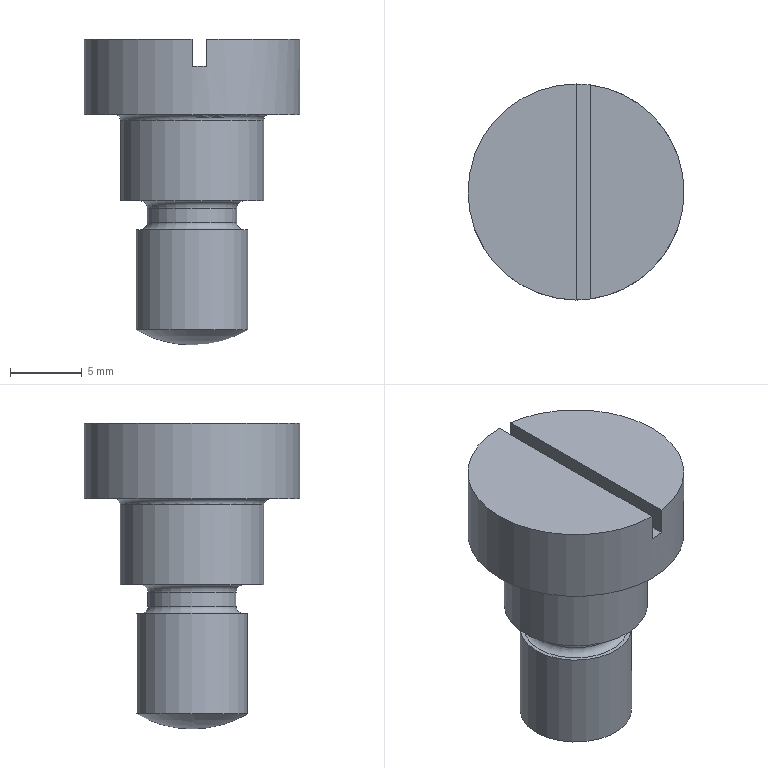Component | NX | GB830-88_M8X6 | 1 solid | 16 faces | box 15 x 15 x 21.24 mm | volume 1783 mm3 | plane 8 | cylinder 4 | torus 3 | sphere 1 | commonest cylinder face diameters 15 x1 9.96 x1 6.2 x1 7.76 x1
STEP:
#1=CARTESIAN_POINT('',(0.,0.,0.));
#2=DIRECTION('',(0.,0.,1.));
#3=DIRECTION('',(1.,0.,0.));
#4=AXIS2_PLACEMENT_3D('',#1,#2,#3);
#5=CARTESIAN_POINT('',(-6.,-7.433,106.24));
#6=VERTEX_POINT('',#5);
#7=CARTESIAN_POINT('',(-6.,7.433,106.24));
#8=VERTEX_POINT('',#7);
#9=CARTESIAN_POINT('',(-6.,-7.5,106.24));
#10=DIRECTION('',(0.,1.,0.));
#11=VECTOR('',#10,1.);
#12=LINE('',#9,#11);
#13=CARTESIAN_POINT('',(0.5,-0.,106.24));
#14=DIRECTION('',(0.,0.,-1.));
#15=DIRECTION('',(-1.,0.,0.));
#16=AXIS2_PLACEMENT_3D('',#13,#14,#15);
#17=PLANE('',#16);
#18=CARTESIAN_POINT('',(6.5,-7.5));
#19=DIRECTION('',(0.,1.));
#20=VECTOR('',#19,1.);
#21=LINE('',#18,#20);
#22=(GEOMETRIC_REPRESENTATION_CONTEXT(2)PARAMETRIC_REPRESENTATION_CONTEXT()REPRESENTATION_CONTEXT('',''));
#23=DEFINITIONAL_REPRESENTATION('',(#21),#22);
#24=PCURVE('',#17,#23);
#25=CARTESIAN_POINT('',(-6.,-7.5,104.34));
#26=DIRECTION('',(-1.,0.,-0.));
#27=DIRECTION('',(-0.,0.,1.));
#28=AXIS2_PLACEMENT_3D('',#25,#26,#27);
#29=PLANE('',#28);
#30=CARTESIAN_POINT('',(1.9,0.));
#31=DIRECTION('',(0.,1.));
#32=VECTOR('',#31,1.);
#33=LINE('',#30,#32);
#34=(GEOMETRIC_REPRESENTATION_CONTEXT(2)PARAMETRIC_REPRESENTATION_CONTEXT()REPRESENTATION_CONTEXT('',''));
#35=DEFINITIONAL_REPRESENTATION('',(#33),#34);
#36=PCURVE('',#29,#35);
#37=SURFACE_CURVE('',#12,(#24,#36),.PCURVE_S1.);
#38=EDGE_CURVE('',#6,#8,#37,.T.);
#39=ORIENTED_EDGE('',*,*,#38,.F.);
#40=CARTESIAN_POINT('',(0.5,-0.,106.24));
#41=VERTEX_POINT('',#40);
#42=CARTESIAN_POINT('',(-7.,-0.,106.24));
#43=DIRECTION('',(0.,0.,1.));
#44=DIRECTION('',(1.,0.,0.));
#45=AXIS2_PLACEMENT_3D('',#42,#43,#44);
#46=CIRCLE('',#45,7.5);
#47=CARTESIAN_POINT('',(0.,0.));
#48=CARTESIAN_POINT('',(0.,12.99));
#49=CARTESIAN_POINT('',(11.25,6.495));
#50=CARTESIAN_POINT('',(22.5,0.));
#51=CARTESIAN_POINT('',(11.25,-6.495));
#52=CARTESIAN_POINT('',(0.,-12.99));
#53=CARTESIAN_POINT('',(0.,0.));
#54=(BOUNDED_CURVE()B_SPLINE_CURVE(2,(#47,#48,#49,#50,#51,#52,#53),.UNSPECIFIED.,.T.,.F.)B_SPLINE_CURVE_WITH_KNOTS((1,2,2,2,2,1),(-2.094,0.,2.094,4.189,6.283,8.378),.UNSPECIFIED.)CURVE()GEOMETRIC_REPRESENTATION_ITEM()RATIONAL_B_SPLINE_CURVE((1.,0.5,1.,0.5,1.,0.5,1.))REPRESENTATION_ITEM(''));
#55=(GEOMETRIC_REPRESENTATION_CONTEXT(2)PARAMETRIC_REPRESENTATION_CONTEXT()REPRESENTATION_CONTEXT('',''));
#56=DEFINITIONAL_REPRESENTATION('',(#54),#55);
#57=PCURVE('',#17,#56);
#58=CARTESIAN_POINT('',(-7.,-0.,101.));
#59=DIRECTION('',(0.,0.,1.));
#60=DIRECTION('',(1.,0.,0.));
#61=AXIS2_PLACEMENT_3D('',#58,#59,#60);
#62=CYLINDRICAL_SURFACE('',#61,7.5);
#63=CARTESIAN_POINT('',(0.,5.24));
#64=DIRECTION('',(1.,0.));
#65=VECTOR('',#64,1.);
#66=LINE('',#63,#65);
#67=(GEOMETRIC_REPRESENTATION_CONTEXT(2)PARAMETRIC_REPRESENTATION_CONTEXT()REPRESENTATION_CONTEXT('',''));
#68=DEFINITIONAL_REPRESENTATION('',(#66),#67);
#69=PCURVE('',#62,#68);
#70=SURFACE_CURVE('',#46,(#57,#69),.PCURVE_S1.);
#71=EDGE_CURVE('',#6,#41,#70,.T.);
#72=ORIENTED_EDGE('',*,*,#71,.T.);
#73=CARTESIAN_POINT('',(-7.,-0.,106.24));
#74=DIRECTION('',(0.,0.,1.));
#75=DIRECTION('',(1.,0.,0.));
#76=AXIS2_PLACEMENT_3D('',#73,#74,#75);
#77=CIRCLE('',#76,7.5);
#78=CARTESIAN_POINT('',(0.,0.));
#79=CARTESIAN_POINT('',(0.,12.99));
#80=CARTESIAN_POINT('',(11.25,6.495));
#81=CARTESIAN_POINT('',(22.5,0.));
#82=CARTESIAN_POINT('',(11.25,-6.495));
#83=CARTESIAN_POINT('',(0.,-12.99));
#84=CARTESIAN_POINT('',(0.,0.));
#85=(BOUNDED_CURVE()B_SPLINE_CURVE(2,(#78,#79,#80,#81,#82,#83,#84),.UNSPECIFIED.,.T.,.F.)B_SPLINE_CURVE_WITH_KNOTS((1,2,2,2,2,1),(-2.094,0.,2.094,4.189,6.283,8.378),.UNSPECIFIED.)CURVE()GEOMETRIC_REPRESENTATION_ITEM()RATIONAL_B_SPLINE_CURVE((1.,0.5,1.,0.5,1.,0.5,1.))REPRESENTATION_ITEM(''));
#86=(GEOMETRIC_REPRESENTATION_CONTEXT(2)PARAMETRIC_REPRESENTATION_CONTEXT()REPRESENTATION_CONTEXT('',''));
#87=DEFINITIONAL_REPRESENTATION('',(#85),#86);
#88=PCURVE('',#17,#87);
#89=CARTESIAN_POINT('',(-6.283,5.24));
#90=DIRECTION('',(1.,0.));
#91=VECTOR('',#90,1.);
#92=LINE('',#89,#91);
#93=(GEOMETRIC_REPRESENTATION_CONTEXT(2)PARAMETRIC_REPRESENTATION_CONTEXT()REPRESENTATION_CONTEXT('',''));
#94=DEFINITIONAL_REPRESENTATION('',(#92),#93);
#95=PCURVE('',#62,#94);
#96=SURFACE_CURVE('',#77,(#88,#95),.PCURVE_S1.);
#97=EDGE_CURVE('',#41,#8,#96,.T.);
#98=ORIENTED_EDGE('',*,*,#97,.T.);
#99=EDGE_LOOP('',(#39,#72,#98));
#100=FACE_BOUND('',#99,.T.);
#101=ADVANCED_FACE('',(#100),#17,.F.);
#102=CARTESIAN_POINT('',(0.5,-0.,101.));
#103=VERTEX_POINT('',#102);
#104=CARTESIAN_POINT('',(-7.,-0.,101.));
#105=DIRECTION('',(0.,0.,1.));
#106=DIRECTION('',(1.,0.,0.));
#107=AXIS2_PLACEMENT_3D('',#104,#105,#106);
#108=CIRCLE('',#107,7.5);
#109=CARTESIAN_POINT('',(0.,0.));
#110=DIRECTION('',(1.,0.));
#111=VECTOR('',#110,1.);
#112=LINE('',#109,#111);
#113=(GEOMETRIC_REPRESENTATION_CONTEXT(2)PARAMETRIC_REPRESENTATION_CONTEXT()REPRESENTATION_CONTEXT('',''));
#114=DEFINITIONAL_REPRESENTATION('',(#112),#113);
#115=PCURVE('',#62,#114);
#116=CARTESIAN_POINT('',(-2.02,-0.,101.));
#117=DIRECTION('',(0.,0.,1.));
#118=DIRECTION('',(1.,0.,0.));
#119=AXIS2_PLACEMENT_3D('',#116,#117,#118);
#120=PLANE('',#119);
#121=CARTESIAN_POINT('',(-4.98,0.));
#122=DIRECTION('',(1.,0.));
#123=AXIS2_PLACEMENT_2D('',#121,#122);
#124=CIRCLE('',#123,7.5);
#125=(GEOMETRIC_REPRESENTATION_CONTEXT(2)PARAMETRIC_REPRESENTATION_CONTEXT()REPRESENTATION_CONTEXT('',''));
#126=DEFINITIONAL_REPRESENTATION('',(#124),#125);
#127=PCURVE('',#120,#126);
#128=SURFACE_CURVE('',#108,(#115,#127),.PCURVE_S1.);
#129=EDGE_CURVE('',#103,#103,#128,.T.);
#130=ORIENTED_EDGE('',*,*,#129,.T.);
#131=CARTESIAN_POINT('',(0.5,-0.,101.));
#132=CARTESIAN_POINT('',(0.5,-0.,106.24));
#133=B_SPLINE_CURVE_WITH_KNOTS('',1,(#131,#132),.UNSPECIFIED.,.F.,.F.,(2,2),(0.,5.24),.PIECEWISE_BEZIER_KNOTS.);
#134=CARTESIAN_POINT('',(6.283,0.));
#135=DIRECTION('',(0.,1.));
#136=VECTOR('',#135,1.);
#137=LINE('',#134,#136);
#138=(GEOMETRIC_REPRESENTATION_CONTEXT(2)PARAMETRIC_REPRESENTATION_CONTEXT()REPRESENTATION_CONTEXT('',''));
#139=DEFINITIONAL_REPRESENTATION('',(#137),#138);
#140=PCURVE('',#62,#139);
#141=CARTESIAN_POINT('',(0.,0.));
#142=DIRECTION('',(0.,1.));
#143=VECTOR('',#142,1.);
#144=LINE('',#141,#143);
#145=(GEOMETRIC_REPRESENTATION_CONTEXT(2)PARAMETRIC_REPRESENTATION_CONTEXT()REPRESENTATION_CONTEXT('',''));
#146=DEFINITIONAL_REPRESENTATION('',(#144),#145);
#147=PCURVE('',#62,#146);
#148=SEAM_CURVE('',#133,(#140,#147),.PCURVE_S1.);
#149=EDGE_CURVE('',#103,#41,#148,.T.);
#150=ORIENTED_EDGE('',*,*,#149,.T.);
#151=ORIENTED_EDGE('',*,*,#71,.F.);
#152=CARTESIAN_POINT('',(-6.,-7.433,104.34));
#153=VERTEX_POINT('',#152);
#154=CARTESIAN_POINT('',(-6.,-7.433,101.));
#155=DIRECTION('',(0.,0.,1.));
#156=VECTOR('',#155,1.);
#157=LINE('',#154,#156);
#158=CARTESIAN_POINT('',(4.846,0.));
#159=DIRECTION('',(0.,1.));
#160=VECTOR('',#159,1.);
#161=LINE('',#158,#160);
#162=(GEOMETRIC_REPRESENTATION_CONTEXT(2)PARAMETRIC_REPRESENTATION_CONTEXT()REPRESENTATION_CONTEXT('',''));
#163=DEFINITIONAL_REPRESENTATION('',(#161),#162);
#164=PCURVE('',#62,#163);
#165=CARTESIAN_POINT('',(-3.34,0.06697));
#166=DIRECTION('',(1.,0.));
#167=VECTOR('',#166,1.);
#168=LINE('',#165,#167);
#169=(GEOMETRIC_REPRESENTATION_CONTEXT(2)PARAMETRIC_REPRESENTATION_CONTEXT()REPRESENTATION_CONTEXT('',''));
#170=DEFINITIONAL_REPRESENTATION('',(#168),#169);
#171=PCURVE('',#29,#170);
#172=SURFACE_CURVE('',#157,(#164,#171),.PCURVE_S1.);
#173=EDGE_CURVE('',#153,#6,#172,.T.);
#174=ORIENTED_EDGE('',*,*,#173,.F.);
#175=CARTESIAN_POINT('',(-7.,-7.5,104.34));
#176=VERTEX_POINT('',#175);
#177=CARTESIAN_POINT('',(-7.,-0.,104.34));
#178=DIRECTION('',(0.,0.,1.));
#179=DIRECTION('',(1.,0.,0.));
#180=AXIS2_PLACEMENT_3D('',#177,#178,#179);
#181=CIRCLE('',#180,7.5);
#182=CARTESIAN_POINT('',(0.,3.34));
#183=DIRECTION('',(1.,0.));
#184=VECTOR('',#183,1.);
#185=LINE('',#182,#184);
#186=(GEOMETRIC_REPRESENTATION_CONTEXT(2)PARAMETRIC_REPRESENTATION_CONTEXT()REPRESENTATION_CONTEXT('',''));
#187=DEFINITIONAL_REPRESENTATION('',(#185),#186);
#188=PCURVE('',#62,#187);
#189=CARTESIAN_POINT('',(-7.,-7.5,104.34));
#190=DIRECTION('',(0.,0.,1.));
#191=DIRECTION('',(1.,0.,0.));
#192=AXIS2_PLACEMENT_3D('',#189,#190,#191);
#193=PLANE('',#192);
#194=CARTESIAN_POINT('',(0.,7.5));
#195=DIRECTION('',(1.,0.));
#196=AXIS2_PLACEMENT_2D('',#194,#195);
#197=CIRCLE('',#196,7.5);
#198=(GEOMETRIC_REPRESENTATION_CONTEXT(2)PARAMETRIC_REPRESENTATION_CONTEXT()REPRESENTATION_CONTEXT('',''));
#199=DEFINITIONAL_REPRESENTATION('',(#197),#198);
#200=PCURVE('',#193,#199);
#201=SURFACE_CURVE('',#181,(#188,#200),.PCURVE_S1.);
#202=EDGE_CURVE('',#176,#153,#201,.T.);
#203=ORIENTED_EDGE('',*,*,#202,.F.);
#204=CARTESIAN_POINT('',(-7.,-7.5,106.24));
#205=VERTEX_POINT('',#204);
#206=CARTESIAN_POINT('',(-7.,-7.5,106.24));
#207=DIRECTION('',(0.,0.,-1.));
#208=VECTOR('',#207,1.);
#209=LINE('',#206,#208);
#210=CARTESIAN_POINT('',(4.712,5.24));
#211=DIRECTION('',(0.,-1.));
#212=VECTOR('',#211,1.);
#213=LINE('',#210,#212);
#214=(GEOMETRIC_REPRESENTATION_CONTEXT(2)PARAMETRIC_REPRESENTATION_CONTEXT()REPRESENTATION_CONTEXT('',''));
#215=DEFINITIONAL_REPRESENTATION('',(#213),#214);
#216=PCURVE('',#62,#215);
#217=CARTESIAN_POINT('',(-7.,-7.5,106.24));
#218=DIRECTION('',(1.,0.,0.));
#219=DIRECTION('',(0.,0.,-1.));
#220=AXIS2_PLACEMENT_3D('',#217,#218,#219);
#221=PLANE('',#220);
#222=CARTESIAN_POINT('',(0.,0.));
#223=DIRECTION('',(1.,0.));
#224=VECTOR('',#223,1.);
#225=LINE('',#222,#224);
#226=(GEOMETRIC_REPRESENTATION_CONTEXT(2)PARAMETRIC_REPRESENTATION_CONTEXT()REPRESENTATION_CONTEXT('',''));
#227=DEFINITIONAL_REPRESENTATION('',(#225),#226);
#228=PCURVE('',#221,#227);
#229=SURFACE_CURVE('',#209,(#216,#228),.PCURVE_S1.);
#230=EDGE_CURVE('',#205,#176,#229,.T.);
#231=ORIENTED_EDGE('',*,*,#230,.F.);
#232=CARTESIAN_POINT('',(-7.,7.5,106.24));
#233=VERTEX_POINT('',#232);
#234=CARTESIAN_POINT('',(-7.,-0.,106.24));
#235=DIRECTION('',(0.,0.,1.));
#236=DIRECTION('',(1.,0.,0.));
#237=AXIS2_PLACEMENT_3D('',#234,#235,#236);
#238=CIRCLE('',#237,7.5);
#239=CARTESIAN_POINT('',(0.,5.24));
#240=DIRECTION('',(1.,0.));
#241=VECTOR('',#240,1.);
#242=LINE('',#239,#241);
#243=(GEOMETRIC_REPRESENTATION_CONTEXT(2)PARAMETRIC_REPRESENTATION_CONTEXT()REPRESENTATION_CONTEXT('',''));
#244=DEFINITIONAL_REPRESENTATION('',(#242),#243);
#245=PCURVE('',#62,#244);
#246=CARTESIAN_POINT('',(0.5,-0.,106.24));
#247=DIRECTION('',(0.,0.,-1.));
#248=DIRECTION('',(-1.,0.,0.));
#249=AXIS2_PLACEMENT_3D('',#246,#247,#248);
#250=PLANE('',#249);
#251=CARTESIAN_POINT('',(0.,0.));
#252=CARTESIAN_POINT('',(0.,12.99));
#253=CARTESIAN_POINT('',(11.25,6.495));
#254=CARTESIAN_POINT('',(22.5,0.));
#255=CARTESIAN_POINT('',(11.25,-6.495));
#256=CARTESIAN_POINT('',(0.,-12.99));
#257=CARTESIAN_POINT('',(0.,0.));
#258=(BOUNDED_CURVE()B_SPLINE_CURVE(2,(#251,#252,#253,#254,#255,#256,#257),.UNSPECIFIED.,.T.,.F.)B_SPLINE_CURVE_WITH_KNOTS((1,2,2,2,2,1),(-2.094,0.,2.094,4.189,6.283,8.378),.UNSPECIFIED.)CURVE()GEOMETRIC_REPRESENTATION_ITEM()RATIONAL_B_SPLINE_CURVE((1.,0.5,1.,0.5,1.,0.5,1.))REPRESENTATION_ITEM(''));
#259=(GEOMETRIC_REPRESENTATION_CONTEXT(2)PARAMETRIC_REPRESENTATION_CONTEXT()REPRESENTATION_CONTEXT('',''));
#260=DEFINITIONAL_REPRESENTATION('',(#258),#259);
#261=PCURVE('',#250,#260);
#262=SURFACE_CURVE('',#238,(#245,#261),.PCURVE_S1.);
#263=EDGE_CURVE('',#233,#205,#262,.T.);
#264=ORIENTED_EDGE('',*,*,#263,.F.);
#265=CARTESIAN_POINT('',(-7.,7.5,104.34));
#266=VERTEX_POINT('',#265);
#267=CARTESIAN_POINT('',(-7.,7.5,106.24));
#268=DIRECTION('',(0.,0.,-1.));
#269=VECTOR('',#268,1.);
#270=LINE('',#267,#269);
#271=CARTESIAN_POINT('',(1.571,5.24));
#272=DIRECTION('',(0.,-1.));
#273=VECTOR('',#272,1.);
#274=LINE('',#271,#273);
#275=(GEOMETRIC_REPRESENTATION_CONTEXT(2)PARAMETRIC_REPRESENTATION_CONTEXT()REPRESENTATION_CONTEXT('',''));
#276=DEFINITIONAL_REPRESENTATION('',(#274),#275);
#277=PCURVE('',#62,#276);
#278=CARTESIAN_POINT('',(0.,15.));
#279=DIRECTION('',(1.,0.));
#280=VECTOR('',#279,1.);
#281=LINE('',#278,#280);
#282=(GEOMETRIC_REPRESENTATION_CONTEXT(2)PARAMETRIC_REPRESENTATION_CONTEXT()REPRESENTATION_CONTEXT('',''));
#283=DEFINITIONAL_REPRESENTATION('',(#281),#282);
#284=PCURVE('',#221,#283);
#285=SURFACE_CURVE('',#270,(#277,#284),.PCURVE_S1.);
#286=EDGE_CURVE('',#233,#266,#285,.T.);
#287=ORIENTED_EDGE('',*,*,#286,.T.);
#288=CARTESIAN_POINT('',(-6.,7.433,104.34));
#289=VERTEX_POINT('',#288);
#290=CARTESIAN_POINT('',(-7.,-0.,104.34));
#291=DIRECTION('',(0.,0.,1.));
#292=DIRECTION('',(1.,0.,0.));
#293=AXIS2_PLACEMENT_3D('',#290,#291,#292);
#294=CIRCLE('',#293,7.5);
#295=CARTESIAN_POINT('',(0.,3.34));
#296=DIRECTION('',(1.,0.));
#297=VECTOR('',#296,1.);
#298=LINE('',#295,#297);
#299=(GEOMETRIC_REPRESENTATION_CONTEXT(2)PARAMETRIC_REPRESENTATION_CONTEXT()REPRESENTATION_CONTEXT('',''));
#300=DEFINITIONAL_REPRESENTATION('',(#298),#299);
#301=PCURVE('',#62,#300);
#302=CARTESIAN_POINT('',(0.,7.5));
#303=DIRECTION('',(1.,0.));
#304=AXIS2_PLACEMENT_2D('',#302,#303);
#305=CIRCLE('',#304,7.5);
#306=(GEOMETRIC_REPRESENTATION_CONTEXT(2)PARAMETRIC_REPRESENTATION_CONTEXT()REPRESENTATION_CONTEXT('',''));
#307=DEFINITIONAL_REPRESENTATION('',(#305),#306);
#308=PCURVE('',#193,#307);
#309=SURFACE_CURVE('',#294,(#301,#308),.PCURVE_S1.);
#310=EDGE_CURVE('',#289,#266,#309,.T.);
#311=ORIENTED_EDGE('',*,*,#310,.F.);
#312=CARTESIAN_POINT('',(-6.,7.433,101.));
#313=DIRECTION('',(0.,0.,-1.));
#314=VECTOR('',#313,1.);
#315=LINE('',#312,#314);
#316=CARTESIAN_POINT('',(1.437,0.));
#317=DIRECTION('',(0.,-1.));
#318=VECTOR('',#317,1.);
#319=LINE('',#316,#318);
#320=(GEOMETRIC_REPRESENTATION_CONTEXT(2)PARAMETRIC_REPRESENTATION_CONTEXT()REPRESENTATION_CONTEXT('',''));
#321=DEFINITIONAL_REPRESENTATION('',(#319),#320);
#322=PCURVE('',#62,#321);
#323=CARTESIAN_POINT('',(-3.34,14.933));
#324=DIRECTION('',(-1.,0.));
#325=VECTOR('',#324,1.);
#326=LINE('',#323,#325);
#327=(GEOMETRIC_REPRESENTATION_CONTEXT(2)PARAMETRIC_REPRESENTATION_CONTEXT()REPRESENTATION_CONTEXT('',''));
#328=DEFINITIONAL_REPRESENTATION('',(#326),#327);
#329=PCURVE('',#29,#328);
#330=SURFACE_CURVE('',#315,(#322,#329),.PCURVE_S1.);
#331=EDGE_CURVE('',#8,#289,#330,.T.);
#332=ORIENTED_EDGE('',*,*,#331,.F.);
#333=ORIENTED_EDGE('',*,*,#97,.F.);
#334=ORIENTED_EDGE('',*,*,#149,.F.);
#335=EDGE_LOOP('',(#130,#150,#151,#174,#203,#231,#264,#287,#311,#332,#333,#334));
#336=FACE_BOUND('',#335,.T.);
#337=ADVANCED_FACE('',(#336),#62,.T.);
#338=ORIENTED_EDGE('',*,*,#263,.T.);
#339=CARTESIAN_POINT('',(-7.,-7.5,106.24));
#340=DIRECTION('',(0.,1.,0.));
#341=VECTOR('',#340,1.);
#342=LINE('',#339,#341);
#343=CARTESIAN_POINT('',(7.5,-7.5));
#344=DIRECTION('',(0.,1.));
#345=VECTOR('',#344,1.);
#346=LINE('',#343,#345);
#347=(GEOMETRIC_REPRESENTATION_CONTEXT(2)PARAMETRIC_REPRESENTATION_CONTEXT()REPRESENTATION_CONTEXT('',''));
#348=DEFINITIONAL_REPRESENTATION('',(#346),#347);
#349=PCURVE('',#250,#348);
#350=CARTESIAN_POINT('',(0.,0.));
#351=DIRECTION('',(0.,1.));
#352=VECTOR('',#351,1.);
#353=LINE('',#350,#352);
#354=(GEOMETRIC_REPRESENTATION_CONTEXT(2)PARAMETRIC_REPRESENTATION_CONTEXT()REPRESENTATION_CONTEXT('',''));
#355=DEFINITIONAL_REPRESENTATION('',(#353),#354);
#356=PCURVE('',#221,#355);
#357=SURFACE_CURVE('',#342,(#349,#356),.PCURVE_S1.);
#358=EDGE_CURVE('',#205,#233,#357,.T.);
#359=ORIENTED_EDGE('',*,*,#358,.T.);
#360=EDGE_LOOP('',(#338,#359));
#361=FACE_BOUND('',#360,.T.);
#362=ADVANCED_FACE('',(#361),#250,.F.);
#363=CARTESIAN_POINT('',(-1.62,-0.,101.));
#364=VERTEX_POINT('',#363);
#365=CARTESIAN_POINT('',(-7.,-0.,101.));
#366=DIRECTION('',(0.,0.,1.));
#367=DIRECTION('',(1.,0.,0.));
#368=AXIS2_PLACEMENT_3D('',#365,#366,#367);
#369=CIRCLE('',#368,5.38);
#370=CARTESIAN_POINT('',(-4.98,0.));
#371=DIRECTION('',(1.,0.));
#372=AXIS2_PLACEMENT_2D('',#370,#371);
#373=CIRCLE('',#372,5.38);
#374=(GEOMETRIC_REPRESENTATION_CONTEXT(2)PARAMETRIC_REPRESENTATION_CONTEXT()REPRESENTATION_CONTEXT('',''));
#375=DEFINITIONAL_REPRESENTATION('',(#373),#374);
#376=PCURVE('',#120,#375);
#377=CARTESIAN_POINT('',(-7.,-0.,100.6));
#378=DIRECTION('',(0.,0.,1.));
#379=DIRECTION('',(1.,0.,0.));
#380=AXIS2_PLACEMENT_3D('',#377,#378,#379);
#381=TOROIDAL_SURFACE('',#380,5.38,0.4);
#382=CARTESIAN_POINT('',(0.,7.854));
#383=DIRECTION('',(1.,0.));
#384=VECTOR('',#383,1.);
#385=LINE('',#382,#384);
#386=(GEOMETRIC_REPRESENTATION_CONTEXT(2)PARAMETRIC_REPRESENTATION_CONTEXT()REPRESENTATION_CONTEXT('',''));
#387=DEFINITIONAL_REPRESENTATION('',(#385),#386);
#388=PCURVE('',#381,#387);
#389=SURFACE_CURVE('',#369,(#376,#388),.PCURVE_S1.);
#390=EDGE_CURVE('',#364,#364,#389,.T.);
#391=ORIENTED_EDGE('',*,*,#390,.T.);
#392=EDGE_LOOP('',(#391));
#393=FACE_BOUND('',#392,.T.);
#394=ORIENTED_EDGE('',*,*,#129,.F.);
#395=EDGE_LOOP('',(#394));
#396=FACE_BOUND('',#395,.T.);
#397=ADVANCED_FACE('',(#393,#396),#120,.F.);
#398=CARTESIAN_POINT('',(-2.02,-0.,100.6));
#399=VERTEX_POINT('',#398);
#400=CARTESIAN_POINT('',(-7.,-0.,100.6));
#401=DIRECTION('',(0.,0.,-1.));
#402=DIRECTION('',(1.,0.,0.));
#403=AXIS2_PLACEMENT_3D('',#400,#401,#402);
#404=CIRCLE('',#403,4.98);
#405=CARTESIAN_POINT('',(-7.,-0.,101.));
#406=DIRECTION('',(0.,0.,1.));
#407=DIRECTION('',(1.,0.,0.));
#408=AXIS2_PLACEMENT_3D('',#405,#406,#407);
#409=CYLINDRICAL_SURFACE('',#408,4.98);
#410=CARTESIAN_POINT('',(6.283,-0.4));
#411=DIRECTION('',(-1.,0.));
#412=VECTOR('',#411,1.);
#413=LINE('',#410,#412);
#414=(GEOMETRIC_REPRESENTATION_CONTEXT(2)PARAMETRIC_REPRESENTATION_CONTEXT()REPRESENTATION_CONTEXT('',''));
#415=DEFINITIONAL_REPRESENTATION('',(#413),#414);
#416=PCURVE('',#409,#415);
#417=CARTESIAN_POINT('',(6.283,9.425));
#418=DIRECTION('',(-1.,0.));
#419=VECTOR('',#418,1.);
#420=LINE('',#417,#419);
#421=(GEOMETRIC_REPRESENTATION_CONTEXT(2)PARAMETRIC_REPRESENTATION_CONTEXT()REPRESENTATION_CONTEXT('',''));
#422=DEFINITIONAL_REPRESENTATION('',(#420),#421);
#423=PCURVE('',#381,#422);
#424=SURFACE_CURVE('',#404,(#416,#423),.PCURVE_S1.);
#425=EDGE_CURVE('',#399,#399,#424,.T.);
#426=ORIENTED_EDGE('',*,*,#425,.T.);
#427=CARTESIAN_POINT('',(-2.02,-0.,95.));
#428=VERTEX_POINT('',#427);
#429=CARTESIAN_POINT('',(-2.02,-0.,95.));
#430=CARTESIAN_POINT('',(-2.02,-0.,100.6));
#431=B_SPLINE_CURVE_WITH_KNOTS('',1,(#429,#430),.UNSPECIFIED.,.F.,.F.,(2,2),(-6.,-0.4),.PIECEWISE_BEZIER_KNOTS.);
#432=CARTESIAN_POINT('',(0.,0.));
#433=DIRECTION('',(0.,1.));
#434=VECTOR('',#433,1.);
#435=LINE('',#432,#434);
#436=(GEOMETRIC_REPRESENTATION_CONTEXT(2)PARAMETRIC_REPRESENTATION_CONTEXT()REPRESENTATION_CONTEXT('',''));
#437=DEFINITIONAL_REPRESENTATION('',(#435),#436);
#438=PCURVE('',#409,#437);
#439=CARTESIAN_POINT('',(6.283,0.));
#440=DIRECTION('',(0.,1.));
#441=VECTOR('',#440,1.);
#442=LINE('',#439,#441);
#443=(GEOMETRIC_REPRESENTATION_CONTEXT(2)PARAMETRIC_REPRESENTATION_CONTEXT()REPRESENTATION_CONTEXT('',''));
#444=DEFINITIONAL_REPRESENTATION('',(#442),#443);
#445=PCURVE('',#409,#444);
#446=SEAM_CURVE('',#431,(#438,#445),.PCURVE_S1.);
#447=EDGE_CURVE('',#428,#399,#446,.T.);
#448=ORIENTED_EDGE('',*,*,#447,.F.);
#449=CARTESIAN_POINT('',(-7.,-0.,95.));
#450=DIRECTION('',(0.,0.,1.));
#451=DIRECTION('',(1.,0.,0.));
#452=AXIS2_PLACEMENT_3D('',#449,#450,#451);
#453=CIRCLE('',#452,4.98);
#454=CARTESIAN_POINT('',(0.,-6.));
#455=DIRECTION('',(1.,0.));
#456=VECTOR('',#455,1.);
#457=LINE('',#454,#456);
#458=(GEOMETRIC_REPRESENTATION_CONTEXT(2)PARAMETRIC_REPRESENTATION_CONTEXT()REPRESENTATION_CONTEXT('',''));
#459=DEFINITIONAL_REPRESENTATION('',(#457),#458);
#460=PCURVE('',#409,#459);
#461=CARTESIAN_POINT('',(-3.9,-0.,95.));
#462=DIRECTION('',(0.,0.,1.));
#463=DIRECTION('',(1.,0.,0.));
#464=AXIS2_PLACEMENT_3D('',#461,#462,#463);
#465=PLANE('',#464);
#466=CARTESIAN_POINT('',(-3.1,0.));
#467=DIRECTION('',(1.,0.));
#468=AXIS2_PLACEMENT_2D('',#466,#467);
#469=CIRCLE('',#468,4.98);
#470=(GEOMETRIC_REPRESENTATION_CONTEXT(2)PARAMETRIC_REPRESENTATION_CONTEXT()REPRESENTATION_CONTEXT('',''));
#471=DEFINITIONAL_REPRESENTATION('',(#469),#470);
#472=PCURVE('',#465,#471);
#473=SURFACE_CURVE('',#453,(#460,#472),.PCURVE_S1.);
#474=EDGE_CURVE('',#428,#428,#473,.T.);
#475=ORIENTED_EDGE('',*,*,#474,.T.);
#476=ORIENTED_EDGE('',*,*,#447,.T.);
#477=EDGE_LOOP('',(#426,#448,#475,#476));
#478=FACE_BOUND('',#477,.T.);
#479=ADVANCED_FACE('',(#478),#409,.T.);
#480=CARTESIAN_POINT('',(-3.4,-0.,95.));
#481=VERTEX_POINT('',#480);
#482=CARTESIAN_POINT('',(-7.,-0.,95.));
#483=DIRECTION('',(0.,0.,1.));
#484=DIRECTION('',(1.,0.,0.));
#485=AXIS2_PLACEMENT_3D('',#482,#483,#484);
#486=CIRCLE('',#485,3.6);
#487=CARTESIAN_POINT('',(-3.1,0.));
#488=DIRECTION('',(1.,0.));
#489=AXIS2_PLACEMENT_2D('',#487,#488);
#490=CIRCLE('',#489,3.6);
#491=(GEOMETRIC_REPRESENTATION_CONTEXT(2)PARAMETRIC_REPRESENTATION_CONTEXT()REPRESENTATION_CONTEXT('',''));
#492=DEFINITIONAL_REPRESENTATION('',(#490),#491);
#493=PCURVE('',#465,#492);
#494=CARTESIAN_POINT('',(-7.,-0.,94.5));
#495=DIRECTION('',(0.,0.,1.));
#496=DIRECTION('',(1.,0.,0.));
#497=AXIS2_PLACEMENT_3D('',#494,#495,#496);
#498=TOROIDAL_SURFACE('',#497,3.6,0.5);
#499=CARTESIAN_POINT('',(0.,7.854));
#500=DIRECTION('',(1.,0.));
#501=VECTOR('',#500,1.);
#502=LINE('',#499,#501);
#503=(GEOMETRIC_REPRESENTATION_CONTEXT(2)PARAMETRIC_REPRESENTATION_CONTEXT()REPRESENTATION_CONTEXT('',''));
#504=DEFINITIONAL_REPRESENTATION('',(#502),#503);
#505=PCURVE('',#498,#504);
#506=SURFACE_CURVE('',#486,(#493,#505),.PCURVE_S1.);
#507=EDGE_CURVE('',#481,#481,#506,.T.);
#508=ORIENTED_EDGE('',*,*,#507,.T.);
#509=EDGE_LOOP('',(#508));
#510=FACE_BOUND('',#509,.T.);
#511=ORIENTED_EDGE('',*,*,#474,.F.);
#512=EDGE_LOOP('',(#511));
#513=FACE_BOUND('',#512,.T.);
#514=ADVANCED_FACE('',(#510,#513),#465,.F.);
#515=CARTESIAN_POINT('',(-10.1,-0.,93.5));
#516=VERTEX_POINT('',#515);
#517=CARTESIAN_POINT('',(-3.9,-0.,93.5));
#518=VERTEX_POINT('',#517);
#519=CARTESIAN_POINT('',(-7.,-0.,93.5));
#520=DIRECTION('',(0.,0.,1.));
#521=DIRECTION('',(-1.,0.,0.));
#522=AXIS2_PLACEMENT_3D('',#519,#520,#521);
#523=CIRCLE('',#522,3.1);
#524=CARTESIAN_POINT('',(-7.,-0.,101.));
#525=DIRECTION('',(0.,0.,1.));
#526=DIRECTION('',(1.,0.,0.));
#527=AXIS2_PLACEMENT_3D('',#524,#525,#526);
#528=CYLINDRICAL_SURFACE('',#527,3.1);
#529=CARTESIAN_POINT('',(3.142,-7.5));
#530=DIRECTION('',(1.,0.));
#531=VECTOR('',#530,1.);
#532=LINE('',#529,#531);
#533=(GEOMETRIC_REPRESENTATION_CONTEXT(2)PARAMETRIC_REPRESENTATION_CONTEXT()REPRESENTATION_CONTEXT('',''));
#534=DEFINITIONAL_REPRESENTATION('',(#532),#533);
#535=PCURVE('',#528,#534);
#536=CARTESIAN_POINT('',(-7.,-0.,93.5));
#537=DIRECTION('',(0.,0.,-1.));
#538=DIRECTION('',(-1.,0.,0.));
#539=AXIS2_PLACEMENT_3D('',#536,#537,#538);
#540=TOROIDAL_SURFACE('',#539,3.6,0.5);
#541=CARTESIAN_POINT('',(6.283,9.425));
#542=DIRECTION('',(-1.,-0.));
#543=VECTOR('',#542,1.);
#544=LINE('',#541,#543);
#545=(GEOMETRIC_REPRESENTATION_CONTEXT(2)PARAMETRIC_REPRESENTATION_CONTEXT()REPRESENTATION_CONTEXT('',''));
#546=DEFINITIONAL_REPRESENTATION('',(#544),#545);
#547=PCURVE('',#540,#546);
#548=SURFACE_CURVE('',#523,(#535,#547),.PCURVE_S1.);
#549=EDGE_CURVE('',#516,#518,#548,.T.);
#550=ORIENTED_EDGE('',*,*,#549,.T.);
#551=CARTESIAN_POINT('',(-3.9,-0.,94.5));
#552=VERTEX_POINT('',#551);
#553=CARTESIAN_POINT('',(-3.9,-0.,93.5));
#554=CARTESIAN_POINT('',(-3.9,-0.,94.5));
#555=B_SPLINE_CURVE_WITH_KNOTS('',1,(#553,#554),.UNSPECIFIED.,.F.,.F.,(2,2),(-7.5,-6.5),.PIECEWISE_BEZIER_KNOTS.);
#556=CARTESIAN_POINT('',(6.283,0.));
#557=DIRECTION('',(0.,1.));
#558=VECTOR('',#557,1.);
#559=LINE('',#556,#558);
#560=(GEOMETRIC_REPRESENTATION_CONTEXT(2)PARAMETRIC_REPRESENTATION_CONTEXT()REPRESENTATION_CONTEXT('',''));
#561=DEFINITIONAL_REPRESENTATION('',(#559),#560);
#562=PCURVE('',#528,#561);
#563=CARTESIAN_POINT('',(0.,0.));
#564=DIRECTION('',(0.,1.));
#565=VECTOR('',#564,1.);
#566=LINE('',#563,#565);
#567=(GEOMETRIC_REPRESENTATION_CONTEXT(2)PARAMETRIC_REPRESENTATION_CONTEXT()REPRESENTATION_CONTEXT('',''));
#568=DEFINITIONAL_REPRESENTATION('',(#566),#567);
#569=PCURVE('',#528,#568);
#570=SEAM_CURVE('',#555,(#562,#569),.PCURVE_S1.);
#571=EDGE_CURVE('',#518,#552,#570,.T.);
#572=ORIENTED_EDGE('',*,*,#571,.T.);
#573=CARTESIAN_POINT('',(-7.,-0.,94.5));
#574=DIRECTION('',(0.,0.,-1.));
#575=DIRECTION('',(1.,0.,0.));
#576=AXIS2_PLACEMENT_3D('',#573,#574,#575);
#577=CIRCLE('',#576,3.1);
#578=CARTESIAN_POINT('',(6.283,-6.5));
#579=DIRECTION('',(-1.,0.));
#580=VECTOR('',#579,1.);
#581=LINE('',#578,#580);
#582=(GEOMETRIC_REPRESENTATION_CONTEXT(2)PARAMETRIC_REPRESENTATION_CONTEXT()REPRESENTATION_CONTEXT('',''));
#583=DEFINITIONAL_REPRESENTATION('',(#581),#582);
#584=PCURVE('',#528,#583);
#585=CARTESIAN_POINT('',(6.283,9.425));
#586=DIRECTION('',(-1.,0.));
#587=VECTOR('',#586,1.);
#588=LINE('',#585,#587);
#589=(GEOMETRIC_REPRESENTATION_CONTEXT(2)PARAMETRIC_REPRESENTATION_CONTEXT()REPRESENTATION_CONTEXT('',''));
#590=DEFINITIONAL_REPRESENTATION('',(#588),#589);
#591=PCURVE('',#498,#590);
#592=SURFACE_CURVE('',#577,(#584,#591),.PCURVE_S1.);
#593=EDGE_CURVE('',#552,#552,#592,.T.);
#594=ORIENTED_EDGE('',*,*,#593,.T.);
#595=ORIENTED_EDGE('',*,*,#571,.F.);
#596=CARTESIAN_POINT('',(-7.,-0.,93.5));
#597=DIRECTION('',(0.,0.,1.));
#598=DIRECTION('',(-1.,0.,0.));
#599=AXIS2_PLACEMENT_3D('',#596,#597,#598);
#600=CIRCLE('',#599,3.1);
#601=CARTESIAN_POINT('',(-3.142,-7.5));
#602=DIRECTION('',(1.,0.));
#603=VECTOR('',#602,1.);
#604=LINE('',#601,#603);
#605=(GEOMETRIC_REPRESENTATION_CONTEXT(2)PARAMETRIC_REPRESENTATION_CONTEXT()REPRESENTATION_CONTEXT('',''));
#606=DEFINITIONAL_REPRESENTATION('',(#604),#605);
#607=PCURVE('',#528,#606);
#608=CARTESIAN_POINT('',(6.283,9.425));
#609=DIRECTION('',(-1.,0.));
#610=VECTOR('',#609,1.);
#611=LINE('',#608,#610);
#612=(GEOMETRIC_REPRESENTATION_CONTEXT(2)PARAMETRIC_REPRESENTATION_CONTEXT()REPRESENTATION_CONTEXT('',''));
#613=DEFINITIONAL_REPRESENTATION('',(#611),#612);
#614=PCURVE('',#540,#613);
#615=SURFACE_CURVE('',#600,(#607,#614),.PCURVE_S1.);
#616=EDGE_CURVE('',#518,#516,#615,.T.);
#617=ORIENTED_EDGE('',*,*,#616,.T.);
#618=EDGE_LOOP('',(#550,#572,#594,#595,#617));
#619=FACE_BOUND('',#618,.T.);
#620=ADVANCED_FACE('',(#619),#528,.T.);
#621=CARTESIAN_POINT('',(-10.6,-0.,93.));
#622=VERTEX_POINT('',#621);
#623=CARTESIAN_POINT('',(-7.,-0.,93.));
#624=DIRECTION('',(0.,0.,-1.));
#625=DIRECTION('',(-1.,0.,0.));
#626=AXIS2_PLACEMENT_3D('',#623,#624,#625);
#627=CIRCLE('',#626,3.6);
#628=CARTESIAN_POINT('',(-3.12,-0.,93.));
#629=DIRECTION('',(0.,0.,-1.));
#630=DIRECTION('',(-1.,0.,0.));
#631=AXIS2_PLACEMENT_3D('',#628,#629,#630);
#632=PLANE('',#631);
#633=CARTESIAN_POINT('',(3.88,0.));
#634=DIRECTION('',(1.,0.));
#635=AXIS2_PLACEMENT_2D('',#633,#634);
#636=CIRCLE('',#635,3.6);
#637=(GEOMETRIC_REPRESENTATION_CONTEXT(2)PARAMETRIC_REPRESENTATION_CONTEXT()REPRESENTATION_CONTEXT('',''));
#638=DEFINITIONAL_REPRESENTATION('',(#636),#637);
#639=PCURVE('',#632,#638);
#640=CARTESIAN_POINT('',(0.,7.854));
#641=DIRECTION('',(1.,0.));
#642=VECTOR('',#641,1.);
#643=LINE('',#640,#642);
#644=(GEOMETRIC_REPRESENTATION_CONTEXT(2)PARAMETRIC_REPRESENTATION_CONTEXT()REPRESENTATION_CONTEXT('',''));
#645=DEFINITIONAL_REPRESENTATION('',(#643),#644);
#646=PCURVE('',#540,#645);
#647=SURFACE_CURVE('',#627,(#639,#646),.PCURVE_S1.);
#648=EDGE_CURVE('',#622,#622,#647,.T.);
#649=ORIENTED_EDGE('',*,*,#648,.T.);
#650=EDGE_LOOP('',(#649));
#651=FACE_BOUND('',#650,.T.);
#652=CARTESIAN_POINT('',(-3.12,-0.,93.));
#653=VERTEX_POINT('',#652);
#654=CARTESIAN_POINT('',(-7.,-0.,93.));
#655=DIRECTION('',(0.,0.,1.));
#656=DIRECTION('',(1.,0.,0.));
#657=AXIS2_PLACEMENT_3D('',#654,#655,#656);
#658=CIRCLE('',#657,3.88);
#659=CARTESIAN_POINT('',(-0.,0.));
#660=CARTESIAN_POINT('',(-0.,6.72));
#661=CARTESIAN_POINT('',(5.82,3.36));
#662=CARTESIAN_POINT('',(11.64,0.));
#663=CARTESIAN_POINT('',(5.82,-3.36));
#664=CARTESIAN_POINT('',(0.,-6.72));
#665=CARTESIAN_POINT('',(-0.,0.));
#666=(BOUNDED_CURVE()B_SPLINE_CURVE(2,(#659,#660,#661,#662,#663,#664,#665),.UNSPECIFIED.,.T.,.F.)B_SPLINE_CURVE_WITH_KNOTS((1,2,2,2,2,1),(-2.094,0.,2.094,4.189,6.283,8.378),.UNSPECIFIED.)CURVE()GEOMETRIC_REPRESENTATION_ITEM()RATIONAL_B_SPLINE_CURVE((1.,0.5,1.,0.5,1.,0.5,1.))REPRESENTATION_ITEM(''));
#667=(GEOMETRIC_REPRESENTATION_CONTEXT(2)PARAMETRIC_REPRESENTATION_CONTEXT()REPRESENTATION_CONTEXT('',''));
#668=DEFINITIONAL_REPRESENTATION('',(#666),#667);
#669=PCURVE('',#632,#668);
#670=CARTESIAN_POINT('',(-7.,-0.,101.));
#671=DIRECTION('',(0.,0.,1.));
#672=DIRECTION('',(1.,0.,0.));
#673=AXIS2_PLACEMENT_3D('',#670,#671,#672);
#674=CYLINDRICAL_SURFACE('',#673,3.88);
#675=CARTESIAN_POINT('',(0.,-8.));
#676=DIRECTION('',(1.,0.));
#677=VECTOR('',#676,1.);
#678=LINE('',#675,#677);
#679=(GEOMETRIC_REPRESENTATION_CONTEXT(2)PARAMETRIC_REPRESENTATION_CONTEXT()REPRESENTATION_CONTEXT('',''));
#680=DEFINITIONAL_REPRESENTATION('',(#678),#679);
#681=PCURVE('',#674,#680);
#682=SURFACE_CURVE('',#658,(#669,#681),.PCURVE_S1.);
#683=EDGE_CURVE('',#653,#653,#682,.T.);
#684=ORIENTED_EDGE('',*,*,#683,.T.);
#685=EDGE_LOOP('',(#684));
#686=FACE_BOUND('',#685,.T.);
#687=ADVANCED_FACE('',(#651,#686),#632,.F.);
#688=ORIENTED_EDGE('',*,*,#683,.F.);
#689=CARTESIAN_POINT('',(-3.12,-0.,86.04));
#690=VERTEX_POINT('',#689);
#691=CARTESIAN_POINT('',(-3.12,-0.,86.04));
#692=CARTESIAN_POINT('',(-3.12,-0.,93.));
#693=B_SPLINE_CURVE_WITH_KNOTS('',1,(#691,#692),.UNSPECIFIED.,.F.,.F.,(2,2),(-14.96,-8.),.PIECEWISE_BEZIER_KNOTS.);
#694=CARTESIAN_POINT('',(0.,0.));
#695=DIRECTION('',(0.,1.));
#696=VECTOR('',#695,1.);
#697=LINE('',#694,#696);
#698=(GEOMETRIC_REPRESENTATION_CONTEXT(2)PARAMETRIC_REPRESENTATION_CONTEXT()REPRESENTATION_CONTEXT('',''));
#699=DEFINITIONAL_REPRESENTATION('',(#697),#698);
#700=PCURVE('',#674,#699);
#701=CARTESIAN_POINT('',(6.283,0.));
#702=DIRECTION('',(0.,1.));
#703=VECTOR('',#702,1.);
#704=LINE('',#701,#703);
#705=(GEOMETRIC_REPRESENTATION_CONTEXT(2)PARAMETRIC_REPRESENTATION_CONTEXT()REPRESENTATION_CONTEXT('',''));
#706=DEFINITIONAL_REPRESENTATION('',(#704),#705);
#707=PCURVE('',#674,#706);
#708=SEAM_CURVE('',#693,(#700,#707),.PCURVE_S1.);
#709=EDGE_CURVE('',#690,#653,#708,.T.);
#710=ORIENTED_EDGE('',*,*,#709,.F.);
#711=CARTESIAN_POINT('',(-10.88,-0.,86.04));
#712=VERTEX_POINT('',#711);
#713=CARTESIAN_POINT('',(-7.,-0.,86.04));
#714=DIRECTION('',(0.,0.,1.));
#715=DIRECTION('',(1.,0.,0.));
#716=AXIS2_PLACEMENT_3D('',#713,#714,#715);
#717=CIRCLE('',#716,3.88);
#718=CARTESIAN_POINT('',(0.,-14.96));
#719=DIRECTION('',(1.,0.));
#720=VECTOR('',#719,1.);
#721=LINE('',#718,#720);
#722=(GEOMETRIC_REPRESENTATION_CONTEXT(2)PARAMETRIC_REPRESENTATION_CONTEXT()REPRESENTATION_CONTEXT('',''));
#723=DEFINITIONAL_REPRESENTATION('',(#721),#722);
#724=PCURVE('',#674,#723);
#725=CARTESIAN_POINT('',(-7.,-0.,92.76));
#726=DIRECTION('',(-0.,0.,1.));
#727=DIRECTION('',(-1.,0.,-0.));
#728=AXIS2_PLACEMENT_3D('',#725,#726,#727);
#729=SPHERICAL_SURFACE('',#728,7.76);
#730=CARTESIAN_POINT('',(3.142,-1.047));
#731=CARTESIAN_POINT('',(3.237,-1.047));
#732=CARTESIAN_POINT('',(3.427,-1.047));
#733=CARTESIAN_POINT('',(3.713,-1.047));
#734=CARTESIAN_POINT('',(3.998,-1.047));
#735=CARTESIAN_POINT('',(4.284,-1.047));
#736=CARTESIAN_POINT('',(4.57,-1.047));
#737=CARTESIAN_POINT('',(4.855,-1.047));
#738=CARTESIAN_POINT('',(5.141,-1.047));
#739=CARTESIAN_POINT('',(5.426,-1.047));
#740=CARTESIAN_POINT('',(5.712,-1.047));
#741=CARTESIAN_POINT('',(5.998,-1.047));
#742=CARTESIAN_POINT('',(6.283,-1.047));
#743=CARTESIAN_POINT('',(6.569,-1.047));
#744=CARTESIAN_POINT('',(6.854,-1.047));
#745=CARTESIAN_POINT('',(7.14,-1.047));
#746=CARTESIAN_POINT('',(7.426,-1.047));
#747=CARTESIAN_POINT('',(7.711,-1.047));
#748=CARTESIAN_POINT('',(7.997,-1.047));
#749=CARTESIAN_POINT('',(8.282,-1.047));
#750=CARTESIAN_POINT('',(8.568,-1.047));
#751=CARTESIAN_POINT('',(8.854,-1.047));
#752=CARTESIAN_POINT('',(9.139,-1.047));
#753=CARTESIAN_POINT('',(9.33,-1.047));
#754=CARTESIAN_POINT('',(9.425,-1.047));
#755=B_SPLINE_CURVE_WITH_KNOTS('',3,(#730,#731,#732,#733,#734,#735,#736,#737,#738,#739,#740,#741,#742,#743,#744,#745,#746,#747,#748,#749,#750,#751,#752,#753,#754),.UNSPECIFIED.,.F.,.F.,(4,1,1,1,1,1,1,1,1,1,1,1,1,1,1,1,1,1,1,1,1,1,4),(0.,0.2856,0.5712,0.8568,1.142,1.428,1.714,1.999,2.285,2.57,2.856,3.142,3.427,3.713,3.998,4.284,4.57,4.855,5.141,5.426,5.712,5.998,6.283),.QUASI_UNIFORM_KNOTS.);
#756=(GEOMETRIC_REPRESENTATION_CONTEXT(2)PARAMETRIC_REPRESENTATION_CONTEXT()REPRESENTATION_CONTEXT('',''));
#757=DEFINITIONAL_REPRESENTATION('',(#755),#756);
#758=PCURVE('',#729,#757);
#759=SURFACE_CURVE('',#717,(#724,#758),.PCURVE_S1.);
#760=EDGE_CURVE('',#690,#712,#759,.T.);
#761=ORIENTED_EDGE('',*,*,#760,.T.);
#762=CARTESIAN_POINT('',(-7.,-0.,86.04));
#763=DIRECTION('',(0.,0.,1.));
#764=DIRECTION('',(1.,0.,0.));
#765=AXIS2_PLACEMENT_3D('',#762,#763,#764);
#766=CIRCLE('',#765,3.88);
#767=CARTESIAN_POINT('',(0.,-14.96));
#768=DIRECTION('',(1.,0.));
#769=VECTOR('',#768,1.);
#770=LINE('',#767,#769);
#771=(GEOMETRIC_REPRESENTATION_CONTEXT(2)PARAMETRIC_REPRESENTATION_CONTEXT()REPRESENTATION_CONTEXT('',''));
#772=DEFINITIONAL_REPRESENTATION('',(#770),#771);
#773=PCURVE('',#674,#772);
#774=CARTESIAN_POINT('',(-3.142,-1.047));
#775=CARTESIAN_POINT('',(-3.046,-1.047));
#776=CARTESIAN_POINT('',(-2.856,-1.047));
#777=CARTESIAN_POINT('',(-2.57,-1.047));
#778=CARTESIAN_POINT('',(-2.285,-1.047));
#779=CARTESIAN_POINT('',(-1.999,-1.047));
#780=CARTESIAN_POINT('',(-1.714,-1.047));
#781=CARTESIAN_POINT('',(-1.428,-1.047));
#782=CARTESIAN_POINT('',(-1.142,-1.047));
#783=CARTESIAN_POINT('',(-0.8568,-1.047));
#784=CARTESIAN_POINT('',(-0.5712,-1.047));
#785=CARTESIAN_POINT('',(-0.2856,-1.047));
#786=CARTESIAN_POINT('',(0.,-1.047));
#787=CARTESIAN_POINT('',(0.2856,-1.047));
#788=CARTESIAN_POINT('',(0.5712,-1.047));
#789=CARTESIAN_POINT('',(0.8568,-1.047));
#790=CARTESIAN_POINT('',(1.142,-1.047));
#791=CARTESIAN_POINT('',(1.428,-1.047));
#792=CARTESIAN_POINT('',(1.714,-1.047));
#793=CARTESIAN_POINT('',(1.999,-1.047));
#794=CARTESIAN_POINT('',(2.285,-1.047));
#795=CARTESIAN_POINT('',(2.57,-1.047));
#796=CARTESIAN_POINT('',(2.856,-1.047));
#797=CARTESIAN_POINT('',(3.046,-1.047));
#798=CARTESIAN_POINT('',(3.142,-1.047));
#799=B_SPLINE_CURVE_WITH_KNOTS('',3,(#774,#775,#776,#777,#778,#779,#780,#781,#782,#783,#784,#785,#786,#787,#788,#789,#790,#791,#792,#793,#794,#795,#796,#797,#798),.UNSPECIFIED.,.F.,.F.,(4,1,1,1,1,1,1,1,1,1,1,1,1,1,1,1,1,1,1,1,1,1,4),(0.,0.2856,0.5712,0.8568,1.142,1.428,1.714,1.999,2.285,2.57,2.856,3.142,3.427,3.713,3.998,4.284,4.57,4.855,5.141,5.426,5.712,5.998,6.283),.QUASI_UNIFORM_KNOTS.);
#800=(GEOMETRIC_REPRESENTATION_CONTEXT(2)PARAMETRIC_REPRESENTATION_CONTEXT()REPRESENTATION_CONTEXT('',''));
#801=DEFINITIONAL_REPRESENTATION('',(#799),#800);
#802=PCURVE('',#729,#801);
#803=SURFACE_CURVE('',#766,(#773,#802),.PCURVE_S1.);
#804=EDGE_CURVE('',#712,#690,#803,.T.);
#805=ORIENTED_EDGE('',*,*,#804,.T.);
#806=ORIENTED_EDGE('',*,*,#709,.T.);
#807=EDGE_LOOP('',(#688,#710,#761,#805,#806));
#808=FACE_BOUND('',#807,.T.);
#809=ADVANCED_FACE('',(#808),#674,.T.);
#810=ORIENTED_EDGE('',*,*,#804,.F.);
#811=CARTESIAN_POINT('',(-7.,-0.,85.));
#812=VERTEX_POINT('',#811);
#813=CARTESIAN_POINT('',(-7.,-0.,85.));
#814=CARTESIAN_POINT('',(-7.813,-0.,85.));
#815=CARTESIAN_POINT('',(-8.625,-0.,85.106));
#816=CARTESIAN_POINT('',(-9.419,-0.,85.319));
#817=CARTESIAN_POINT('',(-10.176,-0.,85.633));
#818=CARTESIAN_POINT('',(-10.88,-0.,86.04));
#819=B_SPLINE_CURVE_WITH_KNOTS('',5,(#813,#814,#815,#816,#817,#818),.UNSPECIFIED.,.F.,.F.,(6,6),(-1.571,-1.047),.PIECEWISE_BEZIER_KNOTS.);
#820=CARTESIAN_POINT('',(0.,0.));
#821=DIRECTION('',(0.,1.));
#822=VECTOR('',#821,1.);
#823=LINE('',#820,#822);
#824=(GEOMETRIC_REPRESENTATION_CONTEXT(2)PARAMETRIC_REPRESENTATION_CONTEXT()REPRESENTATION_CONTEXT('',''));
#825=DEFINITIONAL_REPRESENTATION('',(#823),#824);
#826=PCURVE('',#729,#825);
#827=CARTESIAN_POINT('',(6.283,0.));
#828=DIRECTION('',(0.,1.));
#829=VECTOR('',#828,1.);
#830=LINE('',#827,#829);
#831=(GEOMETRIC_REPRESENTATION_CONTEXT(2)PARAMETRIC_REPRESENTATION_CONTEXT()REPRESENTATION_CONTEXT('',''));
#832=DEFINITIONAL_REPRESENTATION('',(#830),#831);
#833=PCURVE('',#729,#832);
#834=SEAM_CURVE('',#819,(#826,#833),.PCURVE_S1.);
#835=EDGE_CURVE('',#812,#712,#834,.T.);
#836=ORIENTED_EDGE('',*,*,#835,.F.);
#837=ORIENTED_EDGE('',*,*,#835,.T.);
#838=ORIENTED_EDGE('',*,*,#760,.F.);
#839=EDGE_LOOP('',(#810,#836,#837,#838));
#840=FACE_BOUND('',#839,.T.);
#841=ADVANCED_FACE('',(#840),#729,.T.);
#842=ORIENTED_EDGE('',*,*,#173,.T.);
#843=ORIENTED_EDGE('',*,*,#38,.T.);
#844=ORIENTED_EDGE('',*,*,#331,.T.);
#845=CARTESIAN_POINT('',(-6.,-7.5,104.34));
#846=DIRECTION('',(0.,1.,0.));
#847=VECTOR('',#846,1.);
#848=LINE('',#845,#847);
#849=CARTESIAN_POINT('',(0.,0.));
#850=DIRECTION('',(0.,1.));
#851=VECTOR('',#850,1.);
#852=LINE('',#849,#851);
#853=(GEOMETRIC_REPRESENTATION_CONTEXT(2)PARAMETRIC_REPRESENTATION_CONTEXT()REPRESENTATION_CONTEXT('',''));
#854=DEFINITIONAL_REPRESENTATION('',(#852),#853);
#855=PCURVE('',#29,#854);
#856=CARTESIAN_POINT('',(1.,0.));
#857=DIRECTION('',(0.,1.));
#858=VECTOR('',#857,1.);
#859=LINE('',#856,#858);
#860=(GEOMETRIC_REPRESENTATION_CONTEXT(2)PARAMETRIC_REPRESENTATION_CONTEXT()REPRESENTATION_CONTEXT('',''));
#861=DEFINITIONAL_REPRESENTATION('',(#859),#860);
#862=PCURVE('',#193,#861);
#863=SURFACE_CURVE('',#848,(#855,#862),.PCURVE_S1.);
#864=EDGE_CURVE('',#153,#289,#863,.T.);
#865=ORIENTED_EDGE('',*,*,#864,.F.);
#866=EDGE_LOOP('',(#842,#843,#844,#865));
#867=FACE_BOUND('',#866,.T.);
#868=ADVANCED_FACE('',(#867),#29,.T.);
#869=ORIENTED_EDGE('',*,*,#310,.T.);
#870=CARTESIAN_POINT('',(-7.,-7.5,104.34));
#871=DIRECTION('',(0.,1.,0.));
#872=VECTOR('',#871,1.);
#873=LINE('',#870,#872);
#874=CARTESIAN_POINT('',(0.,0.));
#875=DIRECTION('',(0.,1.));
#876=VECTOR('',#875,1.);
#877=LINE('',#874,#876);
#878=(GEOMETRIC_REPRESENTATION_CONTEXT(2)PARAMETRIC_REPRESENTATION_CONTEXT()REPRESENTATION_CONTEXT('',''));
#879=DEFINITIONAL_REPRESENTATION('',(#877),#878);
#880=PCURVE('',#193,#879);
#881=CARTESIAN_POINT('',(1.9,0.));
#882=DIRECTION('',(0.,1.));
#883=VECTOR('',#882,1.);
#884=LINE('',#881,#883);
#885=(GEOMETRIC_REPRESENTATION_CONTEXT(2)PARAMETRIC_REPRESENTATION_CONTEXT()REPRESENTATION_CONTEXT('',''));
#886=DEFINITIONAL_REPRESENTATION('',(#884),#885);
#887=PCURVE('',#221,#886);
#888=SURFACE_CURVE('',#873,(#880,#887),.PCURVE_S1.);
#889=EDGE_CURVE('',#176,#266,#888,.T.);
#890=ORIENTED_EDGE('',*,*,#889,.F.);
#891=ORIENTED_EDGE('',*,*,#202,.T.);
#892=ORIENTED_EDGE('',*,*,#864,.T.);
#893=EDGE_LOOP('',(#869,#890,#891,#892));
#894=FACE_BOUND('',#893,.T.);
#895=ADVANCED_FACE('',(#894),#193,.T.);
#896=ORIENTED_EDGE('',*,*,#286,.F.);
#897=ORIENTED_EDGE('',*,*,#358,.F.);
#898=ORIENTED_EDGE('',*,*,#230,.T.);
#899=ORIENTED_EDGE('',*,*,#889,.T.);
#900=EDGE_LOOP('',(#896,#897,#898,#899));
#901=FACE_BOUND('',#900,.T.);
#902=ADVANCED_FACE('',(#901),#221,.T.);
#903=ORIENTED_EDGE('',*,*,#648,.T.);
#904=CARTESIAN_POINT('',(-10.6,-0.,93.));
#905=CARTESIAN_POINT('',(-10.466,-0.,93.));
#906=CARTESIAN_POINT('',(-10.336,-0.,93.043));
#907=CARTESIAN_POINT('',(-10.224,-0.,93.124));
#908=CARTESIAN_POINT('',(-10.143,-0.,93.236));
#909=CARTESIAN_POINT('',(-10.1,-0.,93.366));
#910=CARTESIAN_POINT('',(-10.1,-0.,93.5));
#911=(BOUNDED_CURVE()B_SPLINE_CURVE(6,(#904,#905,#906,#907,#908,#909,#910),.UNSPECIFIED.,.F.,.F.)B_SPLINE_CURVE_WITH_KNOTS((7,7),(1.571,3.142),.PIECEWISE_BEZIER_KNOTS.)CURVE()GEOMETRIC_REPRESENTATION_ITEM()RATIONAL_B_SPLINE_CURVE((1.031,1.01,0.9979,0.994,0.9979,1.01,1.031))REPRESENTATION_ITEM(''));
#912=CARTESIAN_POINT('',(6.283,6.283));
#913=DIRECTION('',(0.,1.));
#914=VECTOR('',#913,1.);
#915=LINE('',#912,#914);
#916=(GEOMETRIC_REPRESENTATION_CONTEXT(2)PARAMETRIC_REPRESENTATION_CONTEXT()REPRESENTATION_CONTEXT('',''));
#917=DEFINITIONAL_REPRESENTATION('',(#915),#916);
#918=PCURVE('',#540,#917);
#919=CARTESIAN_POINT('',(0.,6.283));
#920=DIRECTION('',(0.,1.));
#921=VECTOR('',#920,1.);
#922=LINE('',#919,#921);
#923=(GEOMETRIC_REPRESENTATION_CONTEXT(2)PARAMETRIC_REPRESENTATION_CONTEXT()REPRESENTATION_CONTEXT('',''));
#924=DEFINITIONAL_REPRESENTATION('',(#922),#923);
#925=PCURVE('',#540,#924);
#926=SEAM_CURVE('',#911,(#918,#925),.PCURVE_S1.);
#927=EDGE_CURVE('',#622,#516,#926,.T.);
#928=ORIENTED_EDGE('',*,*,#927,.T.);
#929=ORIENTED_EDGE('',*,*,#549,.T.);
#930=ORIENTED_EDGE('',*,*,#616,.T.);
#931=ORIENTED_EDGE('',*,*,#927,.F.);
#932=EDGE_LOOP('',(#903,#928,#929,#930,#931));
#933=FACE_BOUND('',#932,.F.);
#934=ADVANCED_FACE('',(#933),#540,.F.);
#935=ORIENTED_EDGE('',*,*,#593,.T.);
#936=CARTESIAN_POINT('',(-3.4,-0.,95.));
#937=CARTESIAN_POINT('',(-3.534,-0.,95.));
#938=CARTESIAN_POINT('',(-3.664,-0.,94.957));
#939=CARTESIAN_POINT('',(-3.776,-0.,94.876));
#940=CARTESIAN_POINT('',(-3.857,-0.,94.764));
#941=CARTESIAN_POINT('',(-3.9,-0.,94.634));
#942=CARTESIAN_POINT('',(-3.9,-0.,94.5));
#943=(BOUNDED_CURVE()B_SPLINE_CURVE(6,(#936,#937,#938,#939,#940,#941,#942),.UNSPECIFIED.,.F.,.F.)B_SPLINE_CURVE_WITH_KNOTS((7,7),(1.571,3.142),.PIECEWISE_BEZIER_KNOTS.)CURVE()GEOMETRIC_REPRESENTATION_ITEM()RATIONAL_B_SPLINE_CURVE((1.031,1.01,0.9979,0.994,0.9979,1.01,1.031))REPRESENTATION_ITEM(''));
#944=CARTESIAN_POINT('',(0.,6.283));
#945=DIRECTION('',(0.,1.));
#946=VECTOR('',#945,1.);
#947=LINE('',#944,#946);
#948=(GEOMETRIC_REPRESENTATION_CONTEXT(2)PARAMETRIC_REPRESENTATION_CONTEXT()REPRESENTATION_CONTEXT('',''));
#949=DEFINITIONAL_REPRESENTATION('',(#947),#948);
#950=PCURVE('',#498,#949);
#951=CARTESIAN_POINT('',(6.283,6.283));
#952=DIRECTION('',(0.,1.));
#953=VECTOR('',#952,1.);
#954=LINE('',#951,#953);
#955=(GEOMETRIC_REPRESENTATION_CONTEXT(2)PARAMETRIC_REPRESENTATION_CONTEXT()REPRESENTATION_CONTEXT('',''));
#956=DEFINITIONAL_REPRESENTATION('',(#954),#955);
#957=PCURVE('',#498,#956);
#958=SEAM_CURVE('',#943,(#950,#957),.PCURVE_S1.);
#959=EDGE_CURVE('',#481,#552,#958,.T.);
#960=ORIENTED_EDGE('',*,*,#959,.F.);
#961=ORIENTED_EDGE('',*,*,#507,.T.);
#962=ORIENTED_EDGE('',*,*,#959,.T.);
#963=EDGE_LOOP('',(#935,#960,#961,#962));
#964=FACE_BOUND('',#963,.F.);
#965=ADVANCED_FACE('',(#964),#498,.F.);
#966=ORIENTED_EDGE('',*,*,#425,.T.);
#967=CARTESIAN_POINT('',(-1.62,-0.,101.));
#968=CARTESIAN_POINT('',(-1.727,-0.,101.));
#969=CARTESIAN_POINT('',(-1.831,-0.,100.966));
#970=CARTESIAN_POINT('',(-1.921,-0.,100.901));
#971=CARTESIAN_POINT('',(-1.986,-0.,100.811));
#972=CARTESIAN_POINT('',(-2.02,-0.,100.707));
#973=CARTESIAN_POINT('',(-2.02,-0.,100.6));
#974=(BOUNDED_CURVE()B_SPLINE_CURVE(6,(#967,#968,#969,#970,#971,#972,#973),.UNSPECIFIED.,.F.,.F.)B_SPLINE_CURVE_WITH_KNOTS((7,7),(1.571,3.142),.PIECEWISE_BEZIER_KNOTS.)CURVE()GEOMETRIC_REPRESENTATION_ITEM()RATIONAL_B_SPLINE_CURVE((1.031,1.01,0.9979,0.994,0.9979,1.01,1.031))REPRESENTATION_ITEM(''));
#975=CARTESIAN_POINT('',(0.,6.283));
#976=DIRECTION('',(0.,1.));
#977=VECTOR('',#976,1.);
#978=LINE('',#975,#977);
#979=(GEOMETRIC_REPRESENTATION_CONTEXT(2)PARAMETRIC_REPRESENTATION_CONTEXT()REPRESENTATION_CONTEXT('',''));
#980=DEFINITIONAL_REPRESENTATION('',(#978),#979);
#981=PCURVE('',#381,#980);
#982=CARTESIAN_POINT('',(6.283,6.283));
#983=DIRECTION('',(0.,1.));
#984=VECTOR('',#983,1.);
#985=LINE('',#982,#984);
#986=(GEOMETRIC_REPRESENTATION_CONTEXT(2)PARAMETRIC_REPRESENTATION_CONTEXT()REPRESENTATION_CONTEXT('',''));
#987=DEFINITIONAL_REPRESENTATION('',(#985),#986);
#988=PCURVE('',#381,#987);
#989=SEAM_CURVE('',#974,(#981,#988),.PCURVE_S1.);
#990=EDGE_CURVE('',#364,#399,#989,.T.);
#991=ORIENTED_EDGE('',*,*,#990,.F.);
#992=ORIENTED_EDGE('',*,*,#390,.T.);
#993=ORIENTED_EDGE('',*,*,#990,.T.);
#994=EDGE_LOOP('',(#966,#991,#992,#993));
#995=FACE_BOUND('',#994,.F.);
#996=ADVANCED_FACE('',(#995),#381,.F.);
#997=CLOSED_SHELL('',(#101,#337,#362,#397,#479,#514,#620,#687,#809,#841,#868,#895,#902,#934,#965,#996));
#998=MANIFOLD_SOLID_BREP('',#997);
#999=(LENGTH_UNIT()NAMED_UNIT(*)SI_UNIT(.MILLI.,.METRE.));
#1000=UNCERTAINTY_MEASURE_WITH_UNIT(LENGTH_MEASURE(0.000005),#999,'','');
#1001=(NAMED_UNIT(*)PLANE_ANGLE_UNIT()SI_UNIT($,.RADIAN.));
#1002=(NAMED_UNIT(*)SI_UNIT($,.STERADIAN.)SOLID_ANGLE_UNIT());
#1003=(GEOMETRIC_REPRESENTATION_CONTEXT(3)GLOBAL_UNCERTAINTY_ASSIGNED_CONTEXT((#1000))GLOBAL_UNIT_ASSIGNED_CONTEXT((#999,#1001,#1002))REPRESENTATION_CONTEXT('',''));
#1004=ADVANCED_BREP_SHAPE_REPRESENTATION('',(#4,#998),#1003);